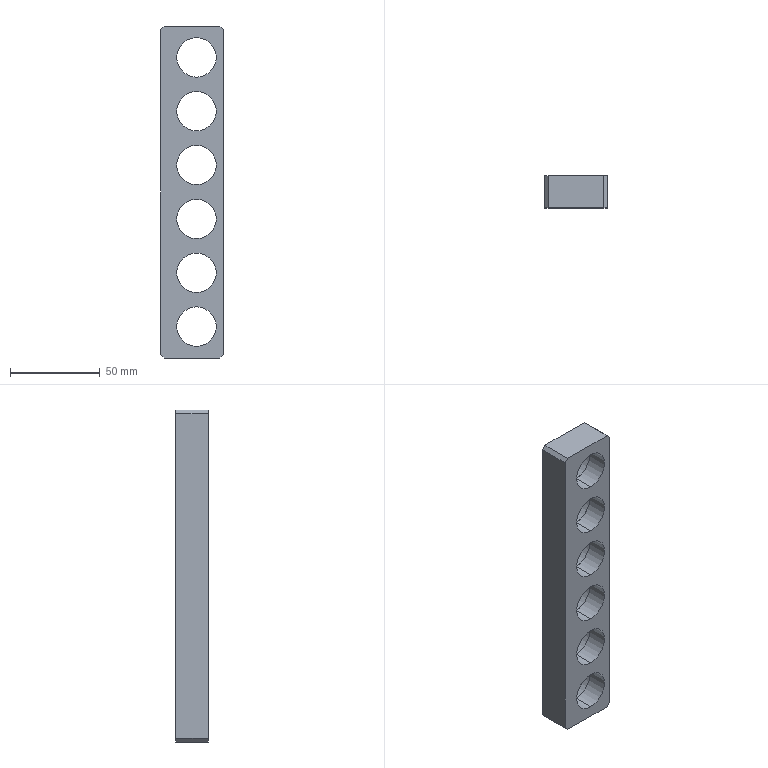Component | SolidWorks | Inline-H010-H01-002K-1 | 1 solid | 88 faces | box 35 x 18 x 185 mm | volume 66413 mm3 | cone 30 | cylinder 30 | plane 28 | commonest cylinder face diameters 28 x18 22 x12
build123d program:
from build123d import *

# Parameters (mm, degrees)
SKETCH1_W           = 185
SKETCH1_H           = 30
BOSS_EXTRUDE1_DEPTH = 9
SKETCH2_R           = 14
CUT_EXTRUDE1_DEPTH  = 6
SKETCH4_R           = 11
CUT_EXTRUDE3_DEPTH  = 95.474
CHAMFER1_SIZE       = 0.5
LPATTERN5_COUNT     = 6
LPATTERN5_PITCH     = 30
CHAMFER2_SIZE       = 0.5
SKETCH5_W           = 8
SKETCH5_H           = 8.652
CUT_EXTRUDE4_DEPTH  = 6
LPATTERN6_COUNT     = 6
LPATTERN6_PITCH     = 30
SKETCH8_W           = 185
SKETCH8_H           = 18
BOSS_EXTRUDE2_DEPTH = 5
CHAMFER3_SIZE       = 2


with BuildPart() as part:
    # Sketch1 → Boss-Extrude1 (new, symmetric)
    with BuildSketch(Plane.XY):
        Rectangle(SKETCH1_W, SKETCH1_H)
    extrude(amount=BOSS_EXTRUDE1_DEPTH, both=True)

    # Sketch2 → Cut-Extrude1 (cut)
    with BuildSketch(Plane.XY.offset(9)):
        with Locations((15, 0)):
            Circle(SKETCH2_R)
        with Locations((-15, 0)):
            Circle(SKETCH2_R)
        with Locations((45, 0)):
            Circle(SKETCH2_R)
        with Locations((75, 0)):
            Circle(SKETCH2_R)
        with Locations((-45, 0)):
            Circle(SKETCH2_R)
        with Locations((-75, 0)):
            Circle(SKETCH2_R)
    extrude(amount=-CUT_EXTRUDE1_DEPTH, mode=Mode.SUBTRACT)

    # Sketch4 → Cut-Extrude3 (cut, through all)
    with BuildSketch(Plane.XY.offset(3)):
        with Locations((75, 0)):
            Circle(SKETCH4_R)
    cut_extrude3 = extrude(amount=-CUT_EXTRUDE3_DEPTH, mode=Mode.SUBTRACT)

    # Chamfer1
    chamfer1_edges = [part.edges().sort_by_distance(p)[0] for p in [
        (61, 0, 9),
        (64, 0, 3),
    ]]
    chamfer(chamfer1_edges, length=CHAMFER1_SIZE)

    # LPattern5: Cut-Extrude3 ×6
    with Locations(*[(-i * LPATTERN5_PITCH, 0, 0) for i in range(1, LPATTERN5_COUNT)]):
        add(cut_extrude3, mode=Mode.SUBTRACT)

    # Chamfer2
    chamfer2_edges = [part.edges().sort_by_distance(p)[0] for p in [
        (1, 0, 9),
        (-29, 0, 9),
        (31, 0, 9),
        (-59, 0, 9),
        (-89, 0, 9),
        (34, 0, 3),
        (4, 0, 3),
        (-26, 0, 3),
        (-56, 0, 3),
        (-86, 0, 3),
    ]]
    chamfer(chamfer2_edges, length=CHAMFER2_SIZE)

    # Sketch5 → Cut-Extrude4 (cut)
    with BuildSketch(Plane.XY.offset(9)):
        with Locations((75, -10.674)):
            Rectangle(SKETCH5_W, SKETCH5_H)
    cut_extrude4 = extrude(amount=-CUT_EXTRUDE4_DEPTH, mode=Mode.SUBTRACT)

    # LPattern6: Cut-Extrude4 ×6
    with Locations(*[(-i * LPATTERN6_PITCH, 0, 0) for i in range(1, LPATTERN6_COUNT)]):
        add(cut_extrude4, mode=Mode.SUBTRACT)

    # Sketch8 → Boss-Extrude2 (add)
    with BuildSketch(Plane(origin=(0, 15, 0), x_dir=(1, 0, 0), z_dir=(0, 1, 0))):
        Rectangle(SKETCH8_W, SKETCH8_H)
    extrude(amount=BOSS_EXTRUDE2_DEPTH)

    # Chamfer3
    chamfer3_edges = [part.edges().sort_by_distance(p)[0] for p in [
        (-92.5, 20, 0),
        (92.5, 20, 0),
        (92.5, -15, 0),
        (-92.5, -15, 0),
    ]]
    chamfer(chamfer3_edges, length=CHAMFER3_SIZE)


solid = part.part

# Placed as in the assembly
solid = solid.moved(Location((29.082, 35.968, 139.665), (-90, 0, 90)))